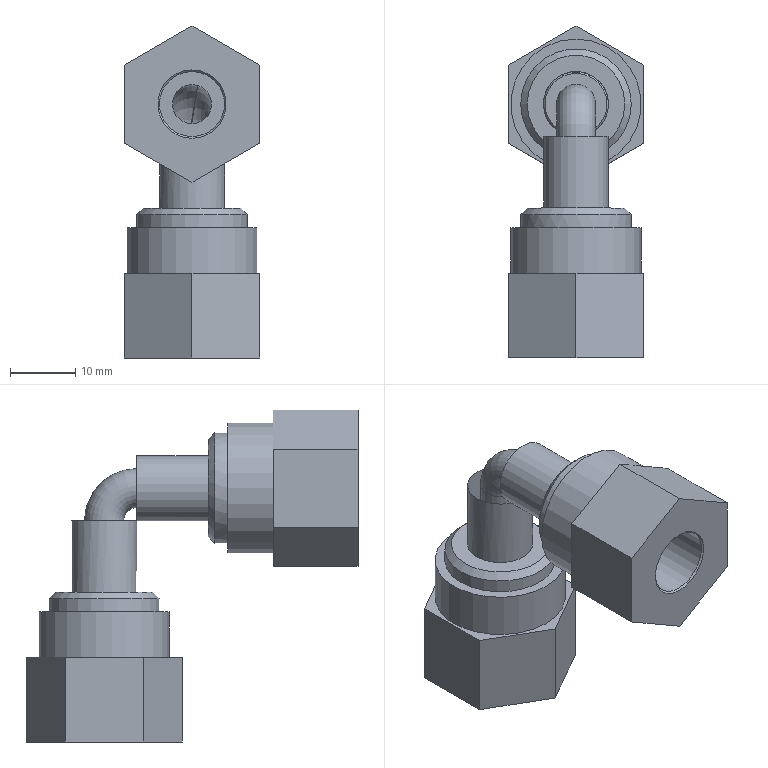Component | NX | CH3404_4-3 | 1 solid | 38 faces | volume 13412 mm3 | plane 22 | cylinder 10 | cone 4 | spline 1 | torus 1 | commonest cylinder face diameters 10 x3 20 x2 17 x2 6 x2 9.5 x1